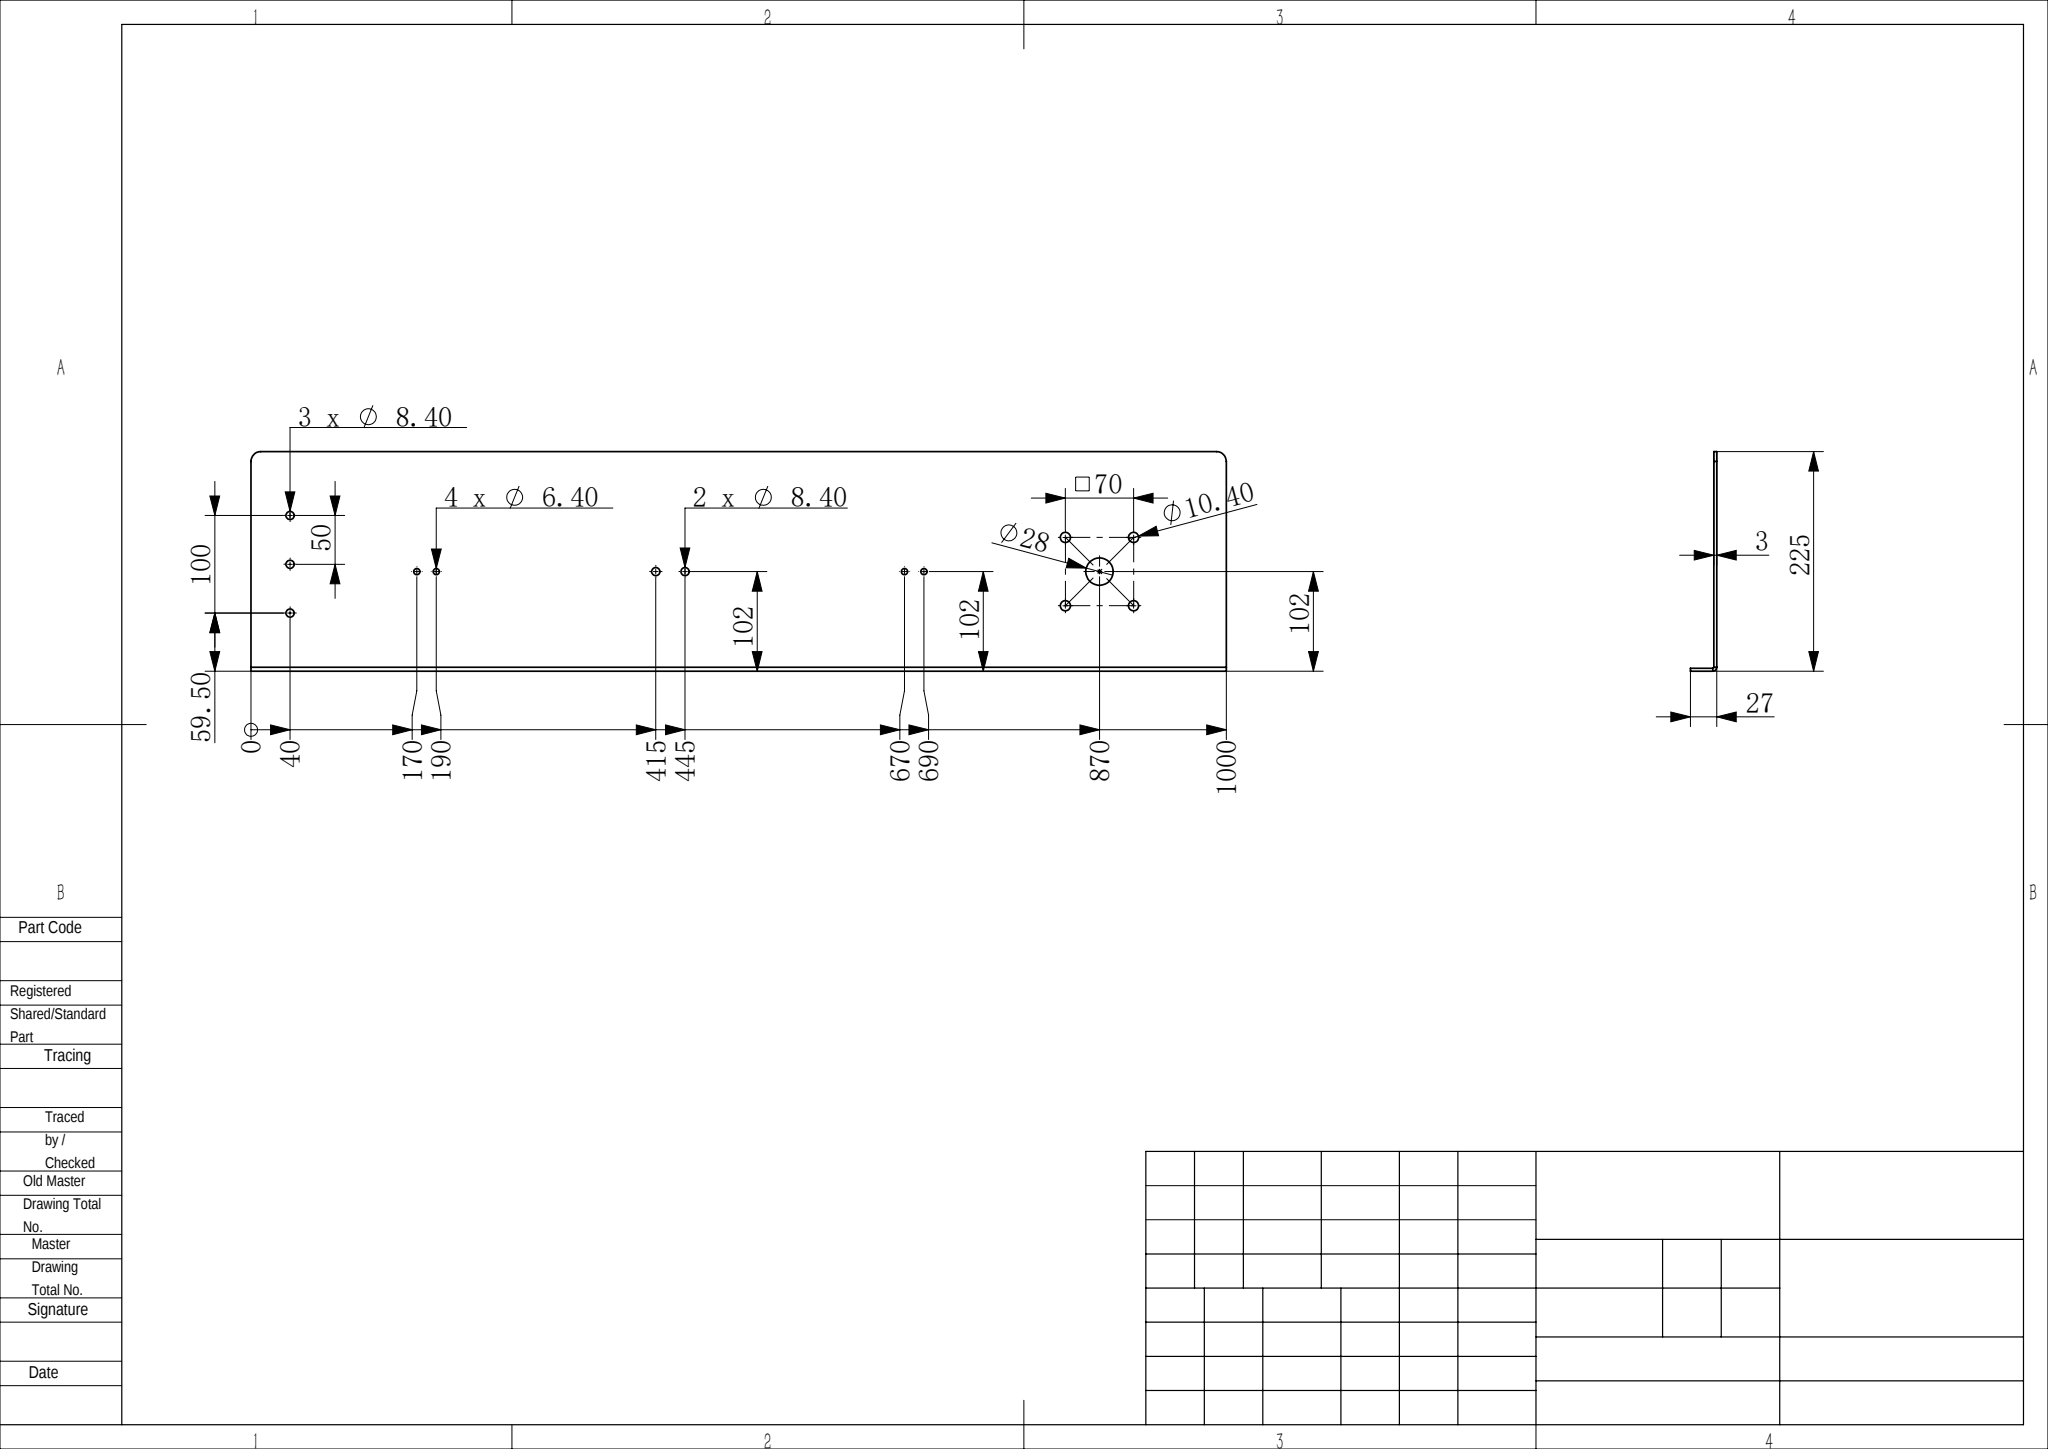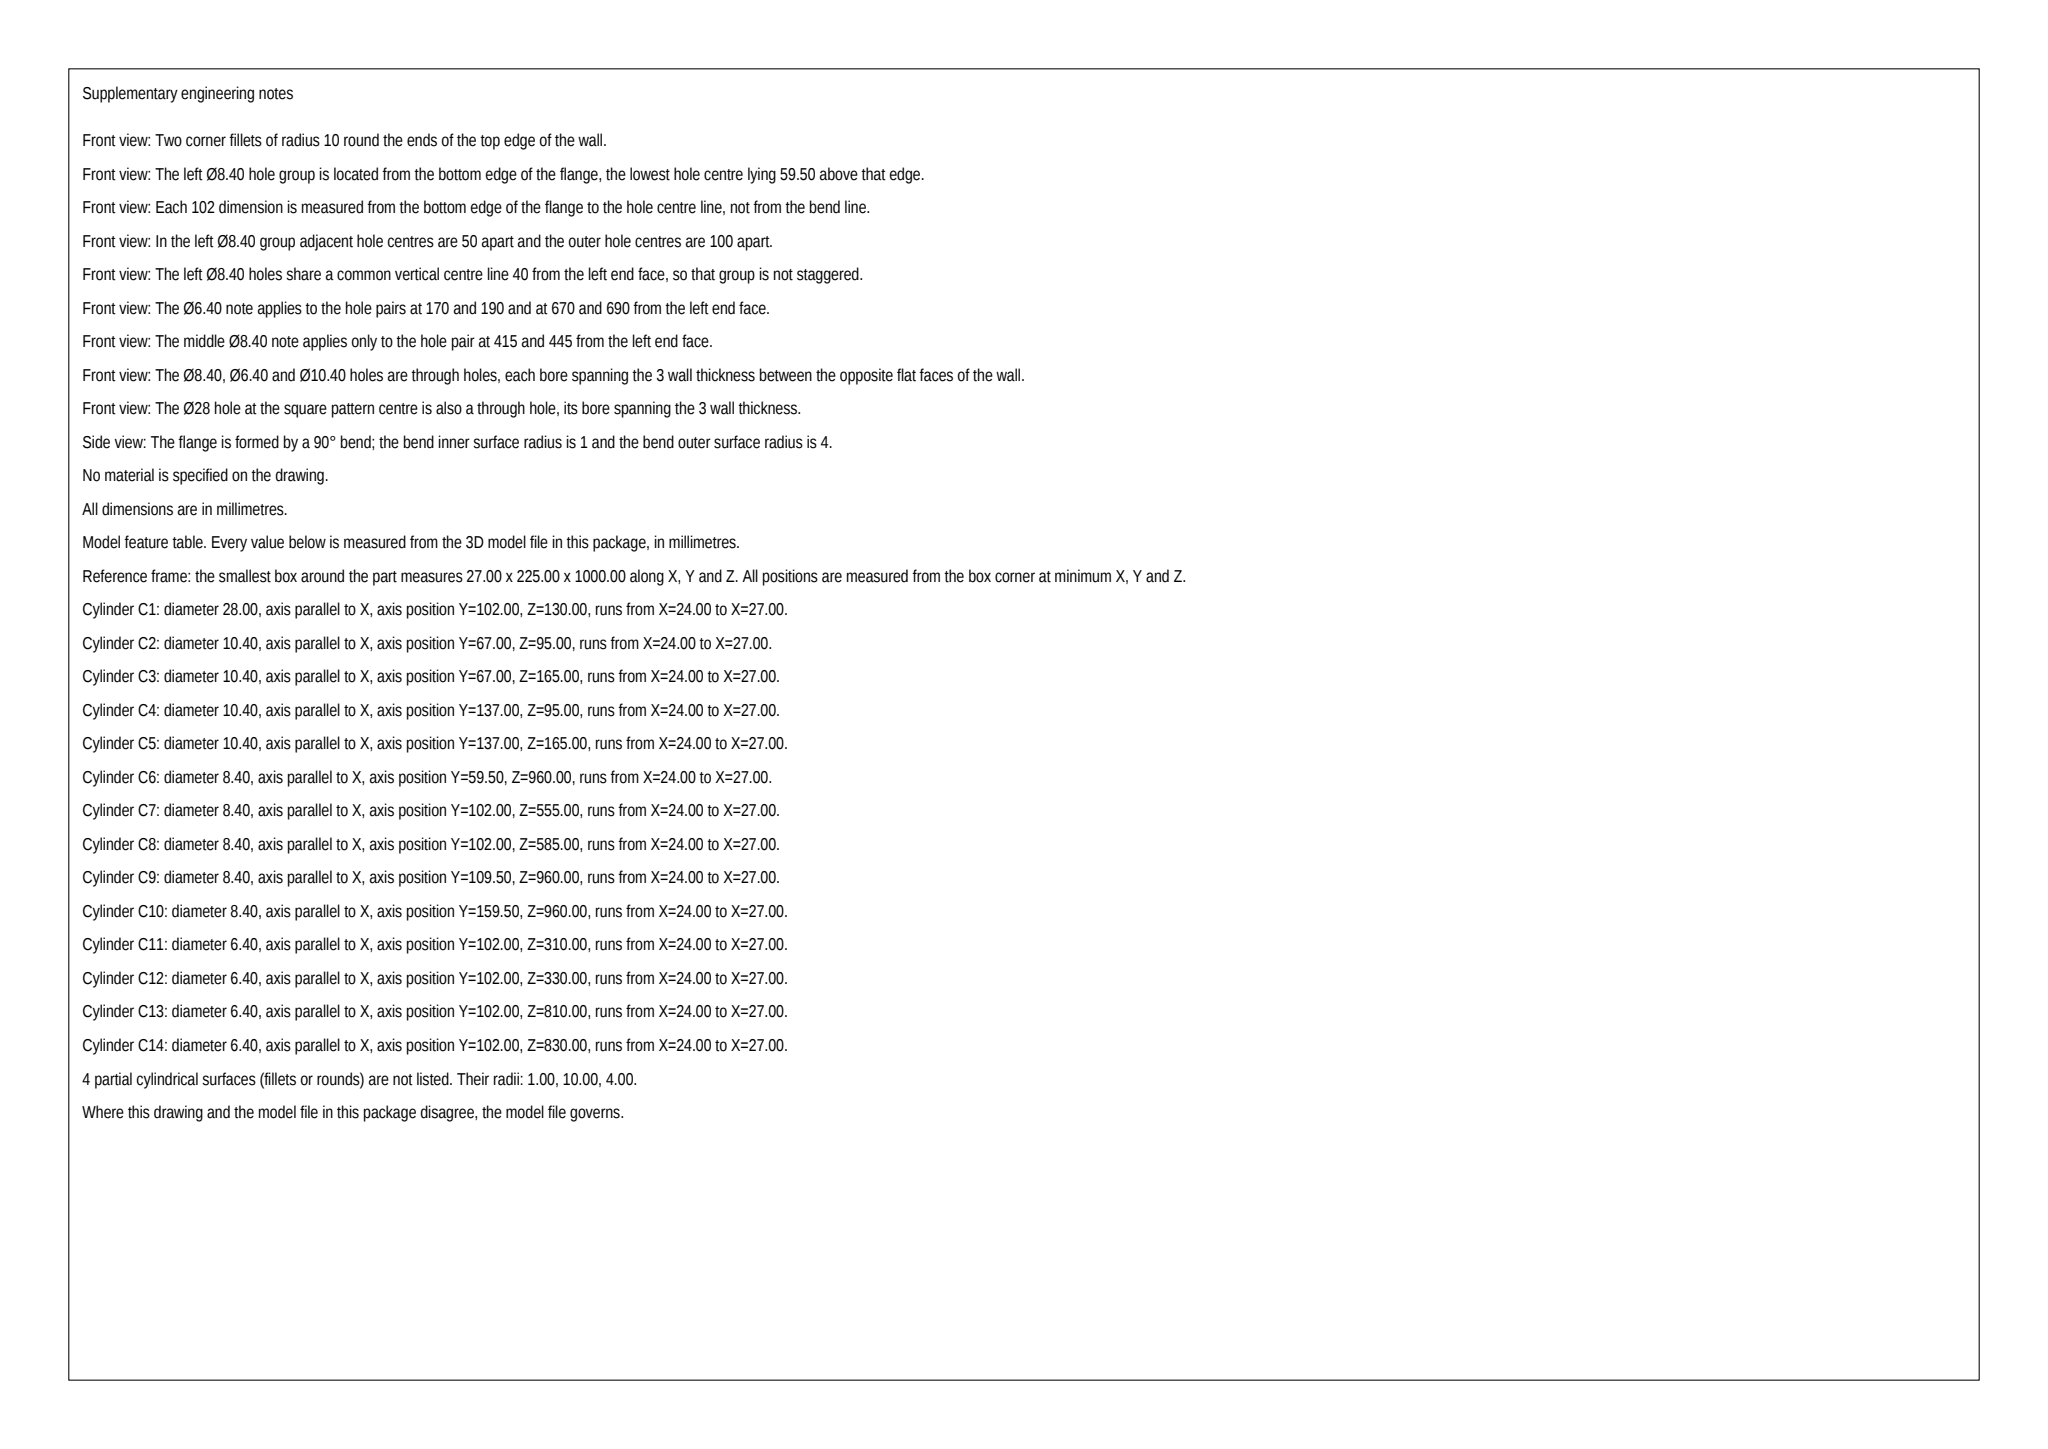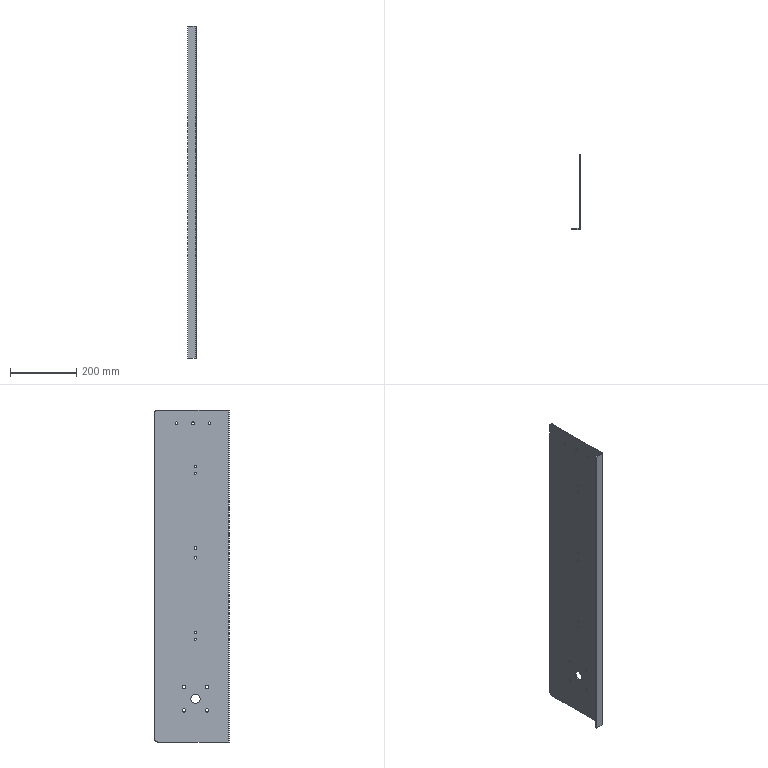Part | SolidWorks | mm | 1 solid | 44 faces | box 27 x 225 x 1000 mm | volume 739568 mm3 | cylinder 32 | plane 12 | commonest cylinder face diameters 8.4 x10 6.4 x8 10.4 x8 28 x2 20 x2 8 x1 2 x1